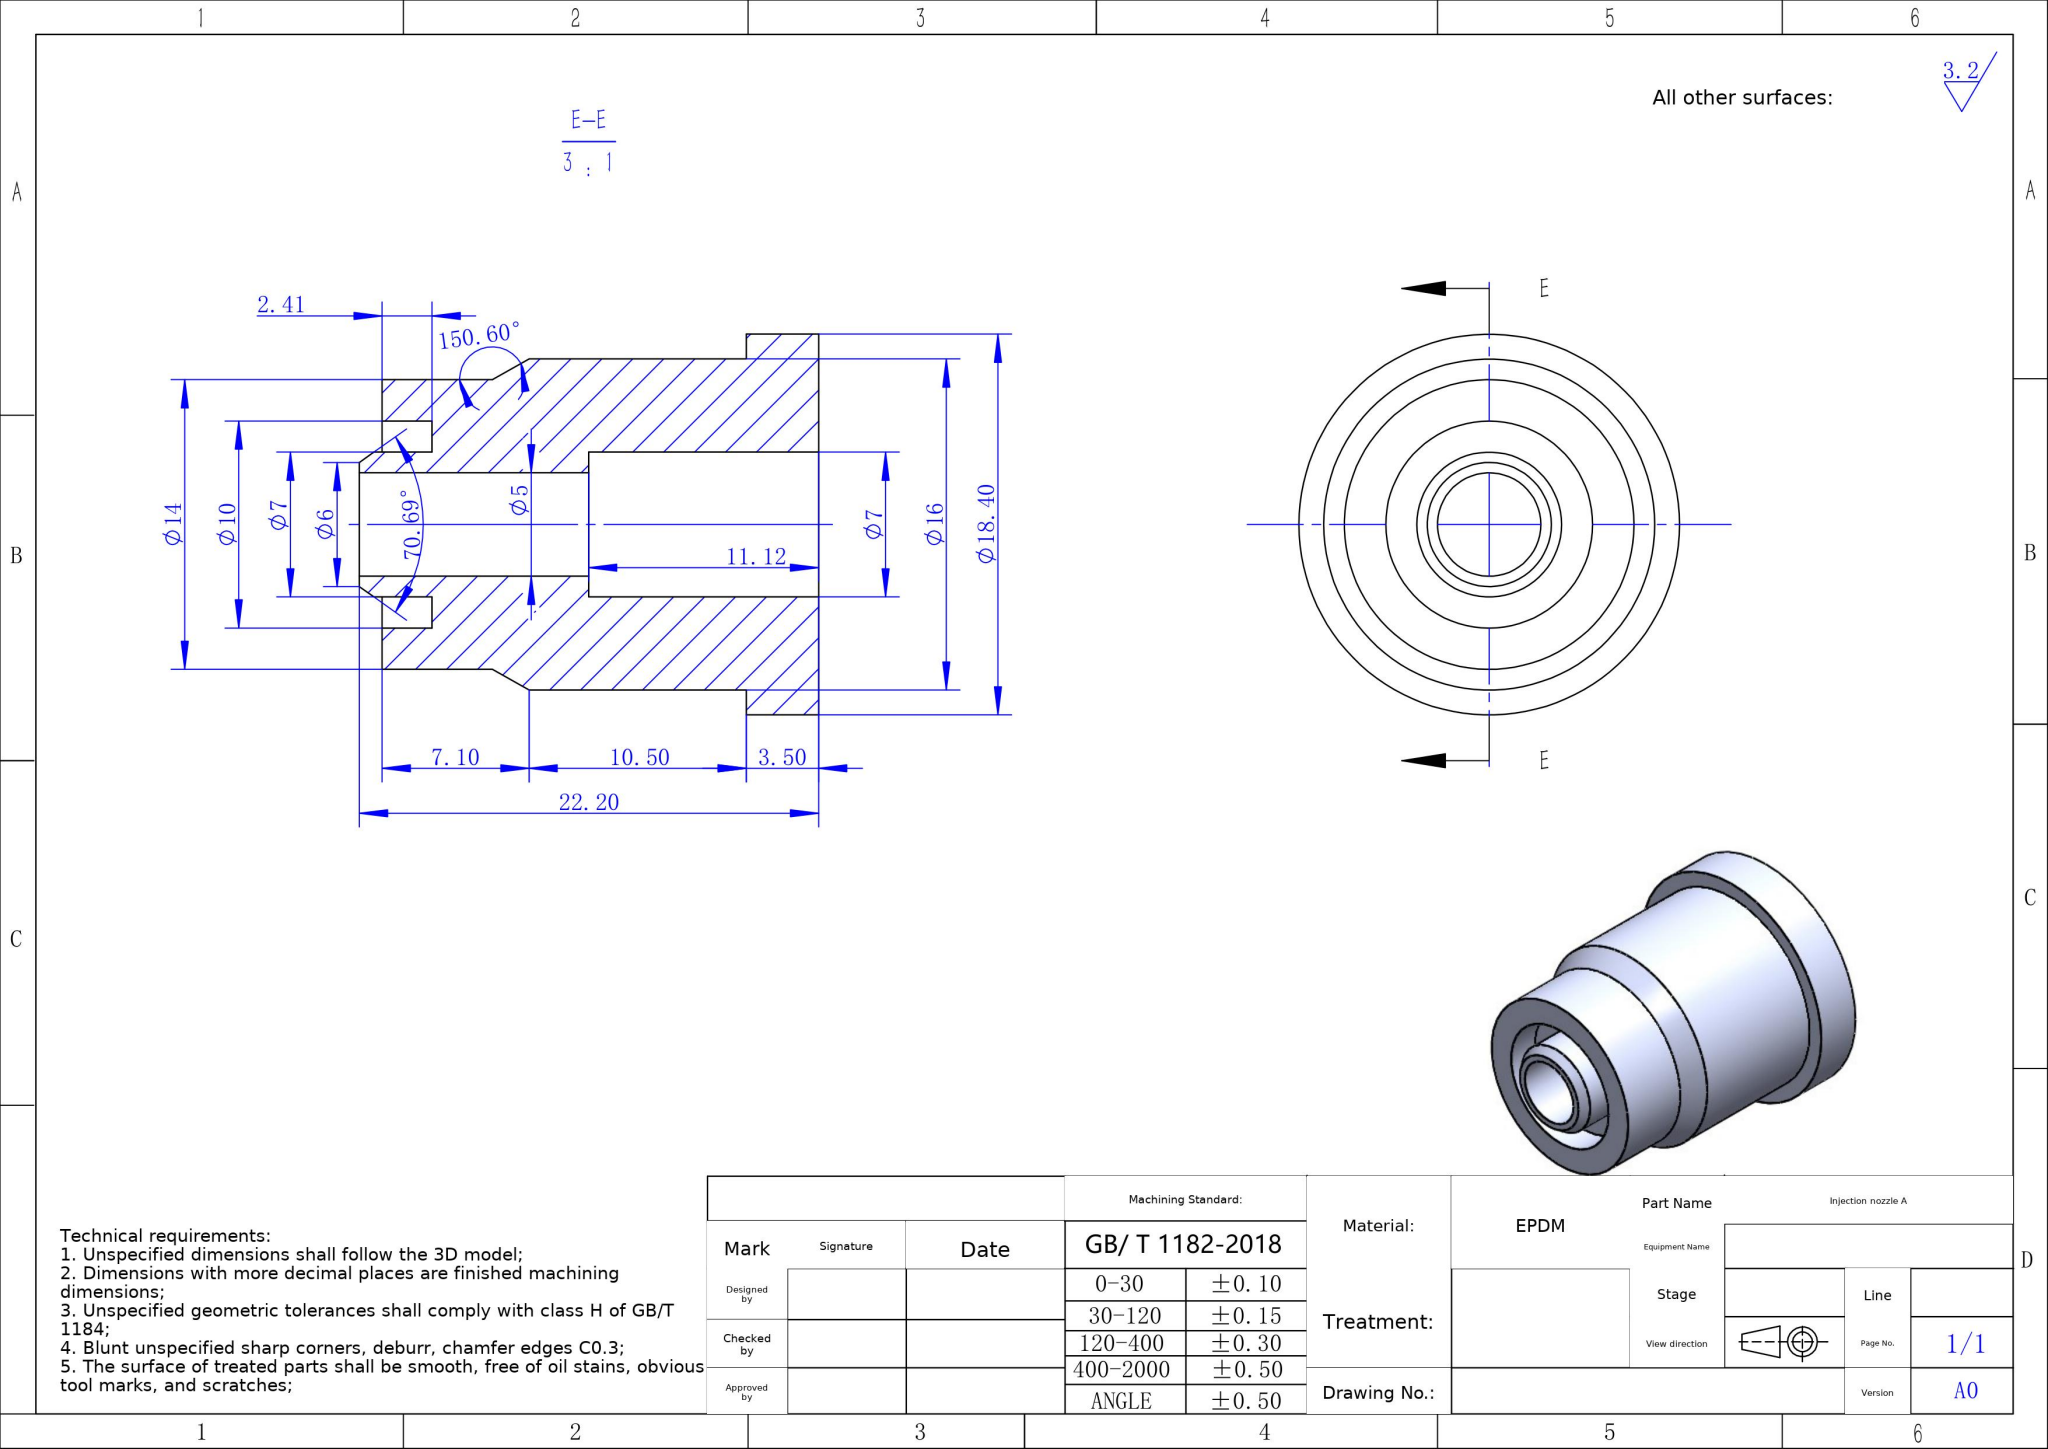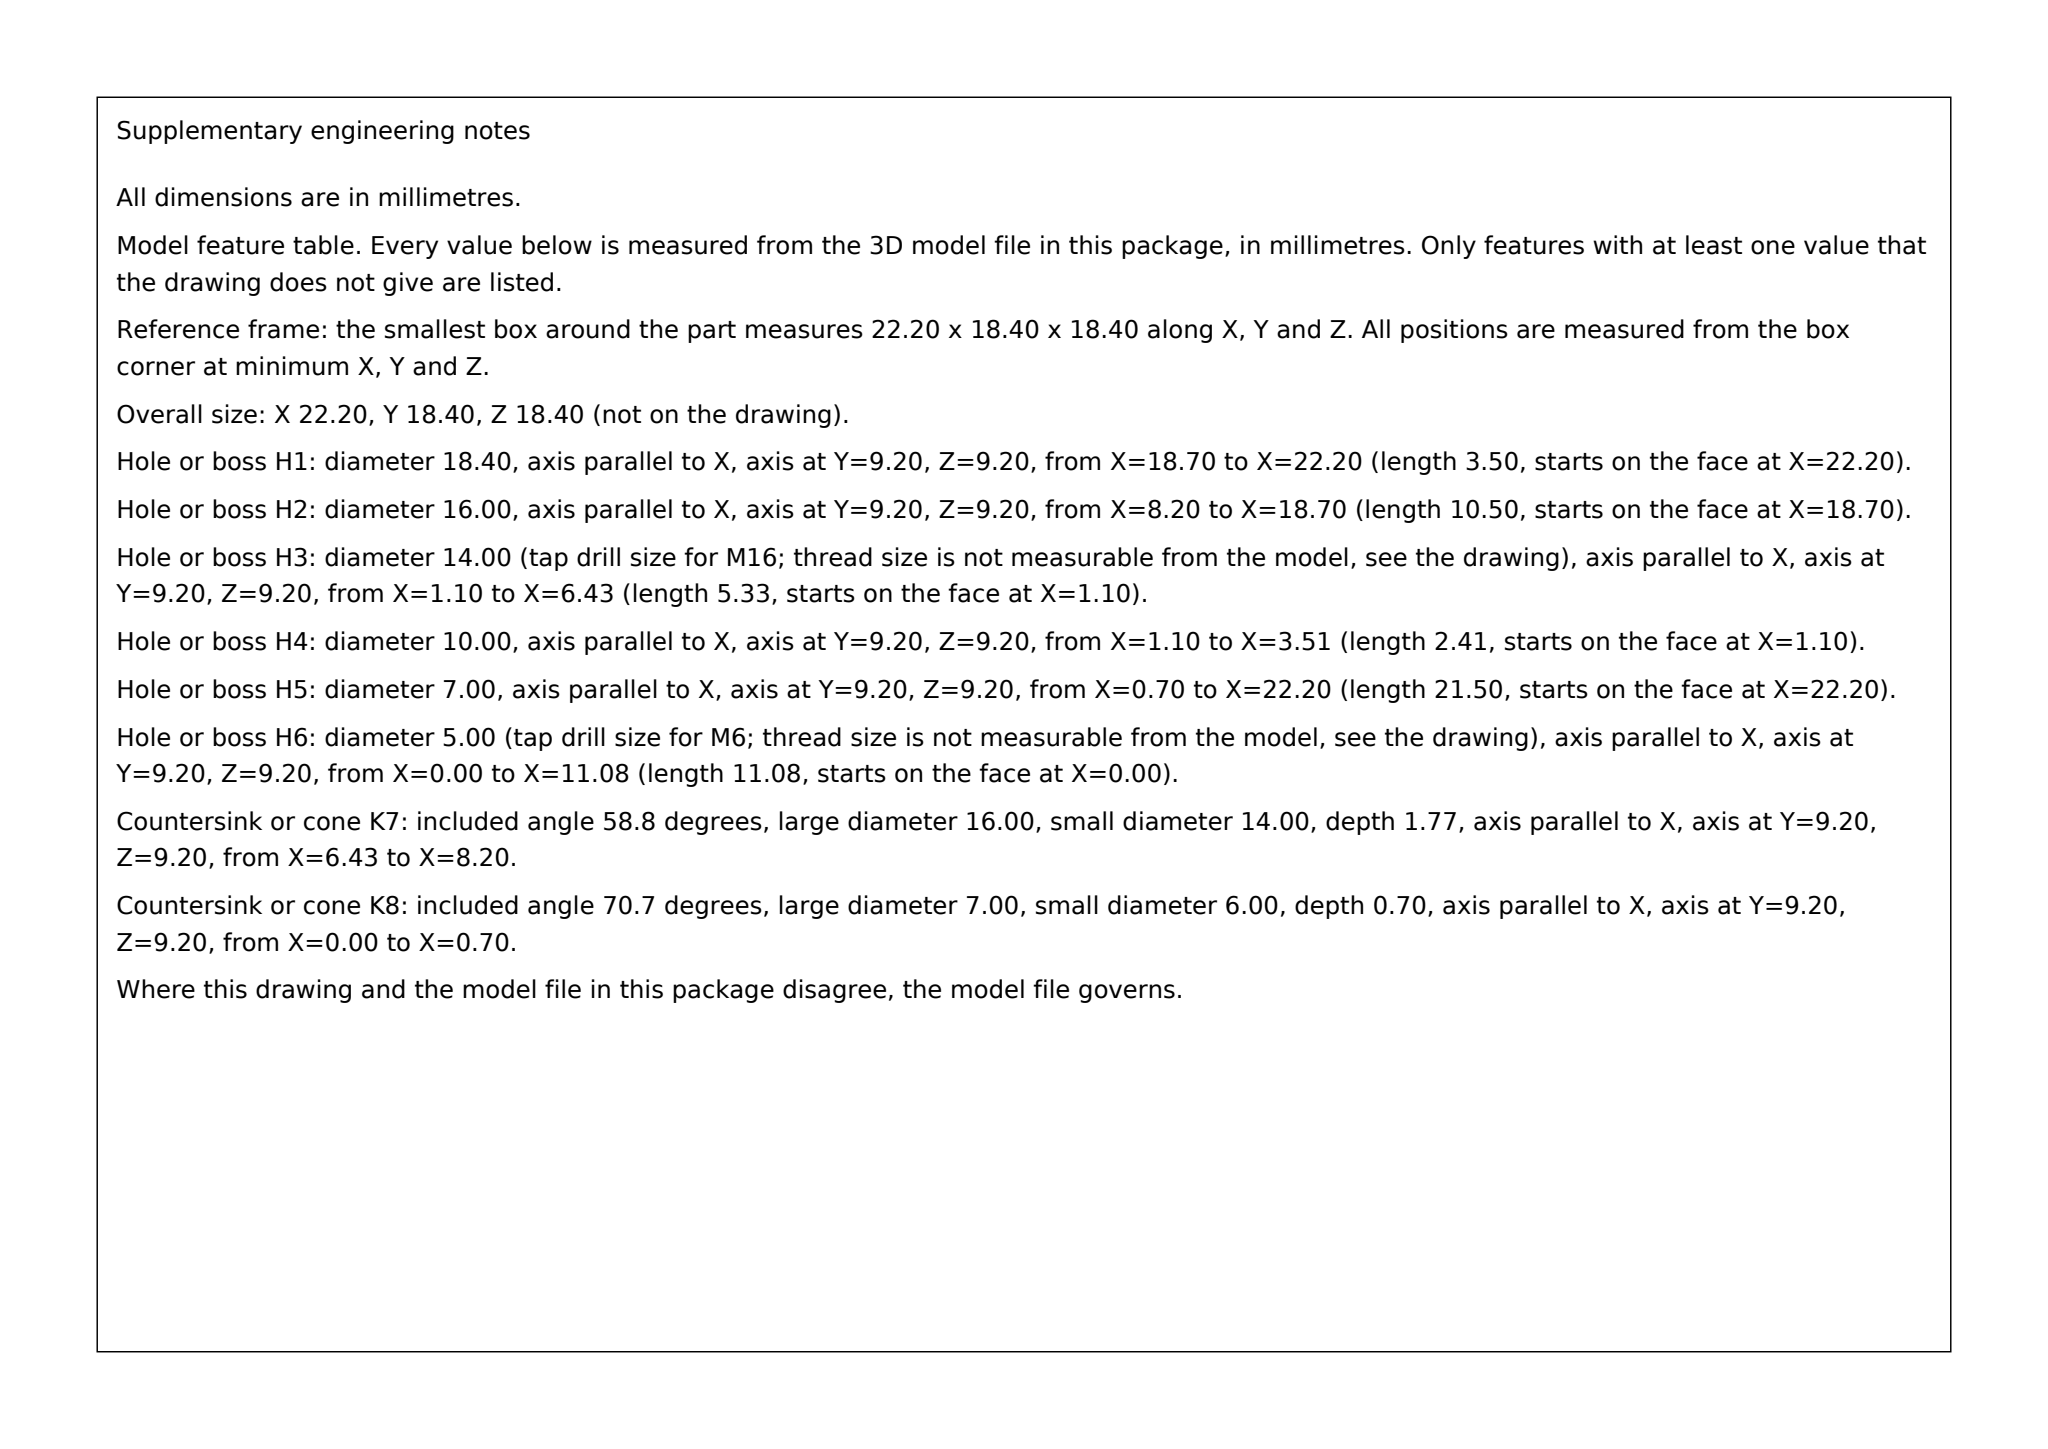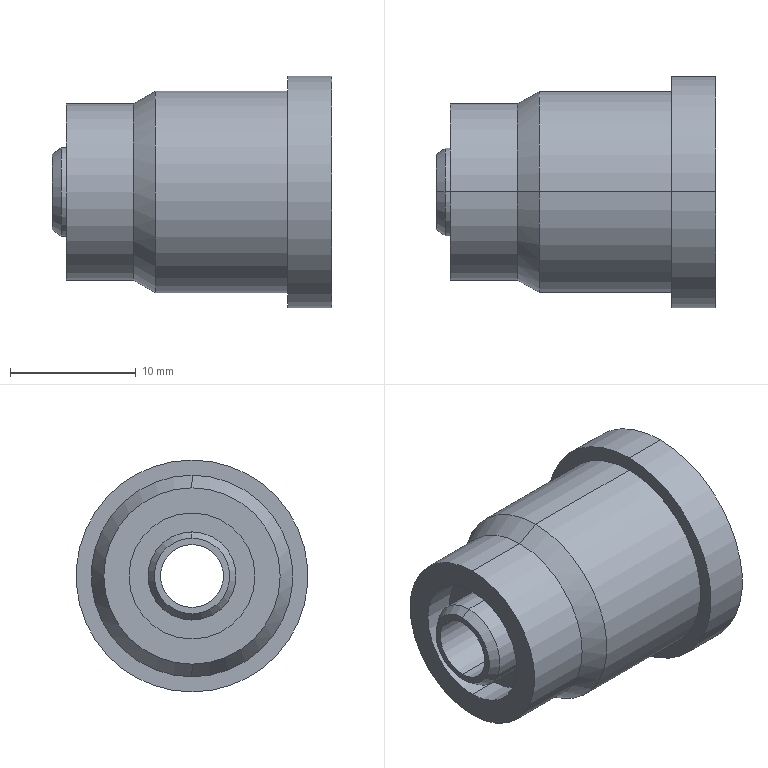Part | SolidWorks | mm | material EPDM | 1 solid | 24 faces | box 22.2 x 18.4 x 18.4 mm | volume 3472 mm3 | cylinder 14 | plane 6 | cone 4 | commonest cylinder face diameters 7 x4 5 x2 10 x2 14 x2 16 x2 18.4 x2
STEP:
#1=CARTESIAN_POINT('',(-32.162,0.,3.));
#2=VERTEX_POINT('',#1);
#3=CARTESIAN_POINT('',(-32.162,0.,-3.));
#4=VERTEX_POINT('',#3);
#5=CARTESIAN_POINT('',(-32.162,0.,0.));
#6=DIRECTION('',(-1.,0.,0.));
#7=DIRECTION('',(0.,0.,1.));
#8=AXIS2_PLACEMENT_3D('',#5,#6,#7);
#9=CIRCLE('',#8,3.);
#10=EDGE_CURVE('',#2,#4,#9,.T.);
#11=ORIENTED_EDGE('',*,*,#10,.F.);
#12=CARTESIAN_POINT('',(-31.457,0.,3.5));
#13=VERTEX_POINT('',#12);
#14=CARTESIAN_POINT('',(-32.162,0.,3.));
#15=DIRECTION('',(0.8157,0.,0.5785));
#16=VECTOR('',#15,1000.);
#17=LINE('',#14,#16);
#18=EDGE_CURVE('',#2,#13,#17,.T.);
#19=ORIENTED_EDGE('',*,*,#18,.T.);
#20=CARTESIAN_POINT('',(-31.457,0.,-3.5));
#21=VERTEX_POINT('',#20);
#22=CARTESIAN_POINT('',(-31.457,0.,0.));
#23=DIRECTION('',(-1.,0.,0.));
#24=DIRECTION('',(0.,0.,-1.));
#25=AXIS2_PLACEMENT_3D('',#22,#23,#24);
#26=CIRCLE('',#25,3.5);
#27=EDGE_CURVE('',#13,#21,#26,.T.);
#28=ORIENTED_EDGE('',*,*,#27,.T.);
#29=CARTESIAN_POINT('',(-32.162,0.,-3.));
#30=DIRECTION('',(0.8157,0.,-0.5785));
#31=VECTOR('',#30,1000.);
#32=LINE('',#29,#31);
#33=EDGE_CURVE('',#4,#21,#32,.T.);
#34=ORIENTED_EDGE('',*,*,#33,.F.);
#35=EDGE_LOOP('',(#11,#19,#28,#34));
#36=FACE_OUTER_BOUND('',#35,.T.);
#37=CARTESIAN_POINT('',(-32.162,0.,0.));
#38=DIRECTION('',(1.,0.,0.));
#39=DIRECTION('',(0.,0.,-1.));
#40=AXIS2_PLACEMENT_3D('',#37,#38,#39);
#41=CONICAL_SURFACE('',#40,3.,0.6169);
#42=ADVANCED_FACE('',(#36),#41,.T.);
#43=CARTESIAN_POINT('',(-9.962,0.,-3.5));
#44=VERTEX_POINT('',#43);
#45=CARTESIAN_POINT('',(-9.962,0.,3.5));
#46=VERTEX_POINT('',#45);
#47=CARTESIAN_POINT('',(-9.962,0.,0.));
#48=DIRECTION('',(-1.,0.,0.));
#49=DIRECTION('',(0.,0.,1.));
#50=AXIS2_PLACEMENT_3D('',#47,#48,#49);
#51=CIRCLE('',#50,3.5);
#52=EDGE_CURVE('',#44,#46,#51,.T.);
#53=ORIENTED_EDGE('',*,*,#52,.F.);
#54=CARTESIAN_POINT('',(-21.082,0.,-3.5));
#55=VERTEX_POINT('',#54);
#56=CARTESIAN_POINT('',(-9.9,0.,-3.5));
#57=DIRECTION('',(-1.,0.,0.));
#58=VECTOR('',#57,1000.);
#59=LINE('',#56,#58);
#60=EDGE_CURVE('',#44,#55,#59,.T.);
#61=ORIENTED_EDGE('',*,*,#60,.T.);
#62=CARTESIAN_POINT('',(-21.082,0.,3.5));
#63=VERTEX_POINT('',#62);
#64=CARTESIAN_POINT('',(-21.082,0.,0.));
#65=DIRECTION('',(-1.,0.,0.));
#66=DIRECTION('',(0.,0.,1.));
#67=AXIS2_PLACEMENT_3D('',#64,#65,#66);
#68=CIRCLE('',#67,3.5);
#69=EDGE_CURVE('',#55,#63,#68,.T.);
#70=ORIENTED_EDGE('',*,*,#69,.T.);
#71=CARTESIAN_POINT('',(-9.9,0.,3.5));
#72=DIRECTION('',(-1.,0.,0.));
#73=VECTOR('',#72,1000.);
#74=LINE('',#71,#73);
#75=EDGE_CURVE('',#46,#63,#74,.T.);
#76=ORIENTED_EDGE('',*,*,#75,.F.);
#77=EDGE_LOOP('',(#53,#61,#70,#76));
#78=FACE_OUTER_BOUND('',#77,.T.);
#79=CARTESIAN_POINT('',(-9.9,0.,0.));
#80=DIRECTION('',(-1.,0.,0.));
#81=DIRECTION('',(0.,0.,1.));
#82=AXIS2_PLACEMENT_3D('',#79,#80,#81);
#83=CYLINDRICAL_SURFACE('',#82,3.5);
#84=ADVANCED_FACE('',(#78),#83,.F.);
#85=CARTESIAN_POINT('',(-21.082,0.,-2.5));
#86=VERTEX_POINT('',#85);
#87=CARTESIAN_POINT('',(-21.082,0.,2.5));
#88=VERTEX_POINT('',#87);
#89=CARTESIAN_POINT('',(-21.082,0.,0.));
#90=DIRECTION('',(-1.,0.,0.));
#91=DIRECTION('',(0.,0.,1.));
#92=AXIS2_PLACEMENT_3D('',#89,#90,#91);
#93=CIRCLE('',#92,2.5);
#94=EDGE_CURVE('',#86,#88,#93,.T.);
#95=ORIENTED_EDGE('',*,*,#94,.F.);
#96=CARTESIAN_POINT('',(-32.162,0.,-2.5));
#97=VERTEX_POINT('',#96);
#98=CARTESIAN_POINT('',(-9.9,0.,-2.5));
#99=DIRECTION('',(-1.,0.,0.));
#100=VECTOR('',#99,1000.);
#101=LINE('',#98,#100);
#102=EDGE_CURVE('',#86,#97,#101,.T.);
#103=ORIENTED_EDGE('',*,*,#102,.T.);
#104=CARTESIAN_POINT('',(-32.162,0.,2.5));
#105=VERTEX_POINT('',#104);
#106=CARTESIAN_POINT('',(-32.162,0.,0.));
#107=DIRECTION('',(-1.,0.,0.));
#108=DIRECTION('',(0.,0.,1.));
#109=AXIS2_PLACEMENT_3D('',#106,#107,#108);
#110=CIRCLE('',#109,2.5);
#111=EDGE_CURVE('',#97,#105,#110,.T.);
#112=ORIENTED_EDGE('',*,*,#111,.T.);
#113=CARTESIAN_POINT('',(-9.9,0.,2.5));
#114=DIRECTION('',(-1.,0.,0.));
#115=VECTOR('',#114,1000.);
#116=LINE('',#113,#115);
#117=EDGE_CURVE('',#88,#105,#116,.T.);
#118=ORIENTED_EDGE('',*,*,#117,.F.);
#119=EDGE_LOOP('',(#95,#103,#112,#118));
#120=FACE_OUTER_BOUND('',#119,.T.);
#121=CARTESIAN_POINT('',(-9.9,0.,0.));
#122=DIRECTION('',(-1.,0.,0.));
#123=DIRECTION('',(0.,0.,1.));
#124=AXIS2_PLACEMENT_3D('',#121,#122,#123);
#125=CYLINDRICAL_SURFACE('',#124,2.5);
#126=ADVANCED_FACE('',(#120),#125,.F.);
#127=CARTESIAN_POINT('',(-28.652,0.,-5.));
#128=VERTEX_POINT('',#127);
#129=CARTESIAN_POINT('',(-28.652,0.,5.));
#130=VERTEX_POINT('',#129);
#131=CARTESIAN_POINT('',(-28.652,0.,0.));
#132=DIRECTION('',(-1.,0.,0.));
#133=DIRECTION('',(0.,0.,1.));
#134=AXIS2_PLACEMENT_3D('',#131,#132,#133);
#135=CIRCLE('',#134,5.);
#136=EDGE_CURVE('',#128,#130,#135,.T.);
#137=ORIENTED_EDGE('',*,*,#136,.F.);
#138=CARTESIAN_POINT('',(-31.062,0.,-5.));
#139=VERTEX_POINT('',#138);
#140=CARTESIAN_POINT('',(-9.9,0.,-5.));
#141=DIRECTION('',(-1.,0.,0.));
#142=VECTOR('',#141,1000.);
#143=LINE('',#140,#142);
#144=EDGE_CURVE('',#128,#139,#143,.T.);
#145=ORIENTED_EDGE('',*,*,#144,.T.);
#146=CARTESIAN_POINT('',(-31.062,0.,5.));
#147=VERTEX_POINT('',#146);
#148=CARTESIAN_POINT('',(-31.062,0.,0.));
#149=DIRECTION('',(-1.,0.,0.));
#150=DIRECTION('',(0.,0.,1.));
#151=AXIS2_PLACEMENT_3D('',#148,#149,#150);
#152=CIRCLE('',#151,5.);
#153=EDGE_CURVE('',#139,#147,#152,.T.);
#154=ORIENTED_EDGE('',*,*,#153,.T.);
#155=CARTESIAN_POINT('',(-9.9,0.,5.));
#156=DIRECTION('',(-1.,0.,0.));
#157=VECTOR('',#156,1000.);
#158=LINE('',#155,#157);
#159=EDGE_CURVE('',#130,#147,#158,.T.);
#160=ORIENTED_EDGE('',*,*,#159,.F.);
#161=EDGE_LOOP('',(#137,#145,#154,#160));
#162=FACE_OUTER_BOUND('',#161,.T.);
#163=CARTESIAN_POINT('',(-9.9,0.,0.));
#164=DIRECTION('',(-1.,0.,0.));
#165=DIRECTION('',(0.,0.,1.));
#166=AXIS2_PLACEMENT_3D('',#163,#164,#165);
#167=CYLINDRICAL_SURFACE('',#166,5.);
#168=ADVANCED_FACE('',(#162),#167,.F.);
#169=CARTESIAN_POINT('',(-25.737,0.,7.));
#170=VERTEX_POINT('',#169);
#171=CARTESIAN_POINT('',(-25.737,0.,-7.));
#172=VERTEX_POINT('',#171);
#173=CARTESIAN_POINT('',(-25.737,0.,0.));
#174=DIRECTION('',(-1.,0.,0.));
#175=DIRECTION('',(0.,0.,1.));
#176=AXIS2_PLACEMENT_3D('',#173,#174,#175);
#177=CIRCLE('',#176,7.);
#178=EDGE_CURVE('',#170,#172,#177,.T.);
#179=ORIENTED_EDGE('',*,*,#178,.T.);
#180=CARTESIAN_POINT('',(-31.062,0.,-7.));
#181=VERTEX_POINT('',#180);
#182=CARTESIAN_POINT('',(-9.9,0.,-7.));
#183=DIRECTION('',(-1.,0.,0.));
#184=VECTOR('',#183,1000.);
#185=LINE('',#182,#184);
#186=EDGE_CURVE('',#172,#181,#185,.T.);
#187=ORIENTED_EDGE('',*,*,#186,.T.);
#188=CARTESIAN_POINT('',(-31.062,0.,7.));
#189=VERTEX_POINT('',#188);
#190=CARTESIAN_POINT('',(-31.062,0.,0.));
#191=DIRECTION('',(-1.,0.,0.));
#192=DIRECTION('',(0.,0.,1.));
#193=AXIS2_PLACEMENT_3D('',#190,#191,#192);
#194=CIRCLE('',#193,7.);
#195=EDGE_CURVE('',#189,#181,#194,.T.);
#196=ORIENTED_EDGE('',*,*,#195,.F.);
#197=CARTESIAN_POINT('',(-9.9,0.,7.));
#198=DIRECTION('',(-1.,0.,0.));
#199=VECTOR('',#198,1000.);
#200=LINE('',#197,#199);
#201=EDGE_CURVE('',#170,#189,#200,.T.);
#202=ORIENTED_EDGE('',*,*,#201,.F.);
#203=EDGE_LOOP('',(#179,#187,#196,#202));
#204=FACE_OUTER_BOUND('',#203,.T.);
#205=CARTESIAN_POINT('',(-9.9,0.,0.));
#206=DIRECTION('',(-1.,0.,0.));
#207=DIRECTION('',(0.,0.,1.));
#208=AXIS2_PLACEMENT_3D('',#205,#206,#207);
#209=CYLINDRICAL_SURFACE('',#208,7.);
#210=ADVANCED_FACE('',(#204),#209,.T.);
#211=ORIENTED_EDGE('',*,*,#178,.F.);
#212=CARTESIAN_POINT('',(-23.962,0.,8.));
#213=VERTEX_POINT('',#212);
#214=CARTESIAN_POINT('',(-23.962,0.,8.));
#215=DIRECTION('',(0.8712,0.,0.4909));
#216=VECTOR('',#215,1000.);
#217=LINE('',#214,#216);
#218=EDGE_CURVE('',#170,#213,#217,.T.);
#219=ORIENTED_EDGE('',*,*,#218,.T.);
#220=CARTESIAN_POINT('',(-23.962,0.,-8.));
#221=VERTEX_POINT('',#220);
#222=CARTESIAN_POINT('',(-23.962,0.,0.));
#223=DIRECTION('',(-1.,0.,0.));
#224=DIRECTION('',(0.,0.,1.));
#225=AXIS2_PLACEMENT_3D('',#222,#223,#224);
#226=CIRCLE('',#225,8.);
#227=EDGE_CURVE('',#213,#221,#226,.T.);
#228=ORIENTED_EDGE('',*,*,#227,.T.);
#229=CARTESIAN_POINT('',(-23.962,0.,-8.));
#230=DIRECTION('',(0.8712,0.,-0.4909));
#231=VECTOR('',#230,1000.);
#232=LINE('',#229,#231);
#233=EDGE_CURVE('',#172,#221,#232,.T.);
#234=ORIENTED_EDGE('',*,*,#233,.F.);
#235=EDGE_LOOP('',(#211,#219,#228,#234));
#236=FACE_OUTER_BOUND('',#235,.T.);
#237=CARTESIAN_POINT('',(-23.962,0.,0.));
#238=DIRECTION('',(1.,0.,0.));
#239=DIRECTION('',(0.,0.,-1.));
#240=AXIS2_PLACEMENT_3D('',#237,#238,#239);
#241=CONICAL_SURFACE('',#240,8.,0.5131);
#242=ADVANCED_FACE('',(#236),#241,.T.);
#243=CARTESIAN_POINT('',(-13.462,0.,8.));
#244=VERTEX_POINT('',#243);
#245=CARTESIAN_POINT('',(-13.462,0.,-8.));
#246=VERTEX_POINT('',#245);
#247=CARTESIAN_POINT('',(-13.462,0.,0.));
#248=DIRECTION('',(-1.,0.,0.));
#249=DIRECTION('',(0.,0.,1.));
#250=AXIS2_PLACEMENT_3D('',#247,#248,#249);
#251=CIRCLE('',#250,8.);
#252=EDGE_CURVE('',#244,#246,#251,.T.);
#253=ORIENTED_EDGE('',*,*,#252,.T.);
#254=CARTESIAN_POINT('',(-9.9,0.,-8.));
#255=DIRECTION('',(-1.,0.,0.));
#256=VECTOR('',#255,1000.);
#257=LINE('',#254,#256);
#258=EDGE_CURVE('',#246,#221,#257,.T.);
#259=ORIENTED_EDGE('',*,*,#258,.T.);
#260=ORIENTED_EDGE('',*,*,#227,.F.);
#261=CARTESIAN_POINT('',(-9.9,0.,8.));
#262=DIRECTION('',(-1.,0.,0.));
#263=VECTOR('',#262,1000.);
#264=LINE('',#261,#263);
#265=EDGE_CURVE('',#244,#213,#264,.T.);
#266=ORIENTED_EDGE('',*,*,#265,.F.);
#267=EDGE_LOOP('',(#253,#259,#260,#266));
#268=FACE_OUTER_BOUND('',#267,.T.);
#269=CARTESIAN_POINT('',(-9.9,0.,0.));
#270=DIRECTION('',(-1.,0.,0.));
#271=DIRECTION('',(0.,0.,1.));
#272=AXIS2_PLACEMENT_3D('',#269,#270,#271);
#273=CYLINDRICAL_SURFACE('',#272,8.);
#274=ADVANCED_FACE('',(#268),#273,.T.);
#275=CARTESIAN_POINT('',(-9.962,0.,9.2));
#276=VERTEX_POINT('',#275);
#277=CARTESIAN_POINT('',(-9.962,0.,-9.2));
#278=VERTEX_POINT('',#277);
#279=CARTESIAN_POINT('',(-9.962,0.,0.));
#280=DIRECTION('',(-1.,0.,0.));
#281=DIRECTION('',(0.,0.,1.));
#282=AXIS2_PLACEMENT_3D('',#279,#280,#281);
#283=CIRCLE('',#282,9.2);
#284=EDGE_CURVE('',#276,#278,#283,.T.);
#285=ORIENTED_EDGE('',*,*,#284,.T.);
#286=CARTESIAN_POINT('',(-13.462,0.,-9.2));
#287=VERTEX_POINT('',#286);
#288=CARTESIAN_POINT('',(-9.9,0.,-9.2));
#289=DIRECTION('',(-1.,0.,0.));
#290=VECTOR('',#289,1000.);
#291=LINE('',#288,#290);
#292=EDGE_CURVE('',#278,#287,#291,.T.);
#293=ORIENTED_EDGE('',*,*,#292,.T.);
#294=CARTESIAN_POINT('',(-13.462,0.,9.2));
#295=VERTEX_POINT('',#294);
#296=CARTESIAN_POINT('',(-13.462,0.,0.));
#297=DIRECTION('',(-1.,0.,0.));
#298=DIRECTION('',(0.,0.,1.));
#299=AXIS2_PLACEMENT_3D('',#296,#297,#298);
#300=CIRCLE('',#299,9.2);
#301=EDGE_CURVE('',#295,#287,#300,.T.);
#302=ORIENTED_EDGE('',*,*,#301,.F.);
#303=CARTESIAN_POINT('',(-9.9,0.,9.2));
#304=DIRECTION('',(-1.,0.,0.));
#305=VECTOR('',#304,1000.);
#306=LINE('',#303,#305);
#307=EDGE_CURVE('',#276,#295,#306,.T.);
#308=ORIENTED_EDGE('',*,*,#307,.F.);
#309=EDGE_LOOP('',(#285,#293,#302,#308));
#310=FACE_OUTER_BOUND('',#309,.T.);
#311=CARTESIAN_POINT('',(-9.9,0.,0.));
#312=DIRECTION('',(-1.,0.,0.));
#313=DIRECTION('',(0.,0.,1.));
#314=AXIS2_PLACEMENT_3D('',#311,#312,#313);
#315=CYLINDRICAL_SURFACE('',#314,9.2);
#316=ADVANCED_FACE('',(#310),#315,.T.);
#317=CARTESIAN_POINT('',(-28.652,0.,3.5));
#318=VERTEX_POINT('',#317);
#319=CARTESIAN_POINT('',(-28.652,0.,-3.5));
#320=VERTEX_POINT('',#319);
#321=CARTESIAN_POINT('',(-28.652,0.,0.));
#322=DIRECTION('',(-1.,0.,0.));
#323=DIRECTION('',(0.,0.,1.));
#324=AXIS2_PLACEMENT_3D('',#321,#322,#323);
#325=CIRCLE('',#324,3.5);
#326=EDGE_CURVE('',#318,#320,#325,.T.);
#327=ORIENTED_EDGE('',*,*,#326,.T.);
#328=CARTESIAN_POINT('',(-9.9,0.,-3.5));
#329=DIRECTION('',(-1.,0.,0.));
#330=VECTOR('',#329,1000.);
#331=LINE('',#328,#330);
#332=EDGE_CURVE('',#320,#21,#331,.T.);
#333=ORIENTED_EDGE('',*,*,#332,.T.);
#334=ORIENTED_EDGE('',*,*,#27,.F.);
#335=CARTESIAN_POINT('',(-9.9,0.,3.5));
#336=DIRECTION('',(-1.,0.,0.));
#337=VECTOR('',#336,1000.);
#338=LINE('',#335,#337);
#339=EDGE_CURVE('',#318,#13,#338,.T.);
#340=ORIENTED_EDGE('',*,*,#339,.F.);
#341=EDGE_LOOP('',(#327,#333,#334,#340));
#342=FACE_OUTER_BOUND('',#341,.T.);
#343=CARTESIAN_POINT('',(-9.9,0.,0.));
#344=DIRECTION('',(-1.,0.,0.));
#345=DIRECTION('',(0.,0.,1.));
#346=AXIS2_PLACEMENT_3D('',#343,#344,#345);
#347=CYLINDRICAL_SURFACE('',#346,3.5);
#348=ADVANCED_FACE('',(#342),#347,.T.);
#349=ORIENTED_EDGE('',*,*,#332,.F.);
#350=CARTESIAN_POINT('',(-28.652,0.,0.));
#351=DIRECTION('',(-1.,0.,0.));
#352=DIRECTION('',(0.,0.,1.));
#353=AXIS2_PLACEMENT_3D('',#350,#351,#352);
#354=CIRCLE('',#353,3.5);
#355=EDGE_CURVE('',#320,#318,#354,.T.);
#356=ORIENTED_EDGE('',*,*,#355,.T.);
#357=ORIENTED_EDGE('',*,*,#339,.T.);
#358=CARTESIAN_POINT('',(-31.457,0.,0.));
#359=DIRECTION('',(-1.,0.,0.));
#360=DIRECTION('',(0.,0.,-1.));
#361=AXIS2_PLACEMENT_3D('',#358,#359,#360);
#362=CIRCLE('',#361,3.5);
#363=EDGE_CURVE('',#21,#13,#362,.T.);
#364=ORIENTED_EDGE('',*,*,#363,.F.);
#365=EDGE_LOOP('',(#349,#356,#357,#364));
#366=FACE_OUTER_BOUND('',#365,.T.);
#367=CARTESIAN_POINT('',(-9.9,0.,0.));
#368=DIRECTION('',(-1.,0.,0.));
#369=DIRECTION('',(0.,0.,1.));
#370=AXIS2_PLACEMENT_3D('',#367,#368,#369);
#371=CYLINDRICAL_SURFACE('',#370,3.5);
#372=ADVANCED_FACE('',(#366),#371,.T.);
#373=CARTESIAN_POINT('',(-32.162,0.,0.));
#374=DIRECTION('',(-1.,0.,0.));
#375=DIRECTION('',(0.,0.,1.));
#376=AXIS2_PLACEMENT_3D('',#373,#374,#375);
#377=CIRCLE('',#376,2.5);
#378=EDGE_CURVE('',#105,#97,#377,.T.);
#379=ORIENTED_EDGE('',*,*,#378,.F.);
#380=ORIENTED_EDGE('',*,*,#111,.F.);
#381=EDGE_LOOP('',(#379,#380));
#382=FACE_BOUND('',#381,.T.);
#383=CARTESIAN_POINT('',(-32.162,0.,0.));
#384=DIRECTION('',(-1.,0.,0.));
#385=DIRECTION('',(0.,0.,1.));
#386=AXIS2_PLACEMENT_3D('',#383,#384,#385);
#387=CIRCLE('',#386,3.);
#388=EDGE_CURVE('',#4,#2,#387,.T.);
#389=ORIENTED_EDGE('',*,*,#388,.T.);
#390=ORIENTED_EDGE('',*,*,#10,.T.);
#391=EDGE_LOOP('',(#389,#390));
#392=FACE_OUTER_BOUND('',#391,.T.);
#393=CARTESIAN_POINT('',(-32.162,3.5,0.));
#394=DIRECTION('',(1.,0.,0.));
#395=DIRECTION('',(0.,0.,-1.));
#396=AXIS2_PLACEMENT_3D('',#393,#394,#395);
#397=PLANE('',#396);
#398=ADVANCED_FACE('',(#382,#392),#397,.F.);
#399=ORIENTED_EDGE('',*,*,#292,.F.);
#400=CARTESIAN_POINT('',(-9.962,0.,0.));
#401=DIRECTION('',(-1.,0.,0.));
#402=DIRECTION('',(0.,0.,1.));
#403=AXIS2_PLACEMENT_3D('',#400,#401,#402);
#404=CIRCLE('',#403,9.2);
#405=EDGE_CURVE('',#278,#276,#404,.T.);
#406=ORIENTED_EDGE('',*,*,#405,.T.);
#407=ORIENTED_EDGE('',*,*,#307,.T.);
#408=CARTESIAN_POINT('',(-13.462,0.,0.));
#409=DIRECTION('',(-1.,0.,0.));
#410=DIRECTION('',(0.,0.,1.));
#411=AXIS2_PLACEMENT_3D('',#408,#409,#410);
#412=CIRCLE('',#411,9.2);
#413=EDGE_CURVE('',#287,#295,#412,.T.);
#414=ORIENTED_EDGE('',*,*,#413,.F.);
#415=EDGE_LOOP('',(#399,#406,#407,#414));
#416=FACE_OUTER_BOUND('',#415,.T.);
#417=CARTESIAN_POINT('',(-9.9,0.,0.));
#418=DIRECTION('',(-1.,0.,0.));
#419=DIRECTION('',(0.,0.,1.));
#420=AXIS2_PLACEMENT_3D('',#417,#418,#419);
#421=CYLINDRICAL_SURFACE('',#420,9.2);
#422=ADVANCED_FACE('',(#416),#421,.T.);
#423=ORIENTED_EDGE('',*,*,#252,.F.);
#424=CARTESIAN_POINT('',(-13.462,0.,0.));
#425=DIRECTION('',(-1.,0.,0.));
#426=DIRECTION('',(0.,0.,1.));
#427=AXIS2_PLACEMENT_3D('',#424,#425,#426);
#428=CIRCLE('',#427,8.);
#429=EDGE_CURVE('',#246,#244,#428,.T.);
#430=ORIENTED_EDGE('',*,*,#429,.F.);
#431=EDGE_LOOP('',(#423,#430));
#432=FACE_BOUND('',#431,.T.);
#433=ORIENTED_EDGE('',*,*,#301,.T.);
#434=ORIENTED_EDGE('',*,*,#413,.T.);
#435=EDGE_LOOP('',(#433,#434));
#436=FACE_OUTER_BOUND('',#435,.T.);
#437=CARTESIAN_POINT('',(-13.462,9.2,0.));
#438=DIRECTION('',(1.,0.,0.));
#439=DIRECTION('',(0.,0.,-1.));
#440=AXIS2_PLACEMENT_3D('',#437,#438,#439);
#441=PLANE('',#440);
#442=ADVANCED_FACE('',(#432,#436),#441,.F.);
#443=ORIENTED_EDGE('',*,*,#258,.F.);
#444=ORIENTED_EDGE('',*,*,#429,.T.);
#445=ORIENTED_EDGE('',*,*,#265,.T.);
#446=CARTESIAN_POINT('',(-23.962,0.,0.));
#447=DIRECTION('',(-1.,0.,0.));
#448=DIRECTION('',(0.,0.,1.));
#449=AXIS2_PLACEMENT_3D('',#446,#447,#448);
#450=CIRCLE('',#449,8.);
#451=EDGE_CURVE('',#221,#213,#450,.T.);
#452=ORIENTED_EDGE('',*,*,#451,.F.);
#453=EDGE_LOOP('',(#443,#444,#445,#452));
#454=FACE_OUTER_BOUND('',#453,.T.);
#455=CARTESIAN_POINT('',(-9.9,0.,0.));
#456=DIRECTION('',(-1.,0.,0.));
#457=DIRECTION('',(0.,0.,1.));
#458=AXIS2_PLACEMENT_3D('',#455,#456,#457);
#459=CYLINDRICAL_SURFACE('',#458,8.);
#460=ADVANCED_FACE('',(#454),#459,.T.);
#461=ORIENTED_EDGE('',*,*,#218,.F.);
#462=CARTESIAN_POINT('',(-25.737,0.,0.));
#463=DIRECTION('',(-1.,0.,0.));
#464=DIRECTION('',(0.,0.,1.));
#465=AXIS2_PLACEMENT_3D('',#462,#463,#464);
#466=CIRCLE('',#465,7.);
#467=EDGE_CURVE('',#172,#170,#466,.T.);
#468=ORIENTED_EDGE('',*,*,#467,.F.);
#469=ORIENTED_EDGE('',*,*,#233,.T.);
#470=ORIENTED_EDGE('',*,*,#451,.T.);
#471=EDGE_LOOP('',(#461,#468,#469,#470));
#472=FACE_OUTER_BOUND('',#471,.T.);
#473=CARTESIAN_POINT('',(-23.962,0.,0.));
#474=DIRECTION('',(1.,0.,0.));
#475=DIRECTION('',(0.,0.,-1.));
#476=AXIS2_PLACEMENT_3D('',#473,#474,#475);
#477=CONICAL_SURFACE('',#476,8.,0.5131);
#478=ADVANCED_FACE('',(#472),#477,.T.);
#479=ORIENTED_EDGE('',*,*,#186,.F.);
#480=ORIENTED_EDGE('',*,*,#467,.T.);
#481=ORIENTED_EDGE('',*,*,#201,.T.);
#482=CARTESIAN_POINT('',(-31.062,0.,0.));
#483=DIRECTION('',(-1.,0.,0.));
#484=DIRECTION('',(0.,0.,1.));
#485=AXIS2_PLACEMENT_3D('',#482,#483,#484);
#486=CIRCLE('',#485,7.);
#487=EDGE_CURVE('',#181,#189,#486,.T.);
#488=ORIENTED_EDGE('',*,*,#487,.F.);
#489=EDGE_LOOP('',(#479,#480,#481,#488));
#490=FACE_OUTER_BOUND('',#489,.T.);
#491=CARTESIAN_POINT('',(-9.9,0.,0.));
#492=DIRECTION('',(-1.,0.,0.));
#493=DIRECTION('',(0.,0.,1.));
#494=AXIS2_PLACEMENT_3D('',#491,#492,#493);
#495=CYLINDRICAL_SURFACE('',#494,7.);
#496=ADVANCED_FACE('',(#490),#495,.T.);
#497=CARTESIAN_POINT('',(-31.062,0.,0.));
#498=DIRECTION('',(-1.,0.,0.));
#499=DIRECTION('',(0.,0.,1.));
#500=AXIS2_PLACEMENT_3D('',#497,#498,#499);
#501=CIRCLE('',#500,5.);
#502=EDGE_CURVE('',#147,#139,#501,.T.);
#503=ORIENTED_EDGE('',*,*,#502,.F.);
#504=ORIENTED_EDGE('',*,*,#153,.F.);
#505=EDGE_LOOP('',(#503,#504));
#506=FACE_BOUND('',#505,.T.);
#507=ORIENTED_EDGE('',*,*,#195,.T.);
#508=ORIENTED_EDGE('',*,*,#487,.T.);
#509=EDGE_LOOP('',(#507,#508));
#510=FACE_OUTER_BOUND('',#509,.T.);
#511=CARTESIAN_POINT('',(-31.062,7.,0.));
#512=DIRECTION('',(1.,0.,0.));
#513=DIRECTION('',(0.,0.,-1.));
#514=AXIS2_PLACEMENT_3D('',#511,#512,#513);
#515=PLANE('',#514);
#516=ADVANCED_FACE('',(#506,#510),#515,.F.);
#517=ORIENTED_EDGE('',*,*,#144,.F.);
#518=CARTESIAN_POINT('',(-28.652,0.,0.));
#519=DIRECTION('',(-1.,0.,0.));
#520=DIRECTION('',(0.,0.,1.));
#521=AXIS2_PLACEMENT_3D('',#518,#519,#520);
#522=CIRCLE('',#521,5.);
#523=EDGE_CURVE('',#130,#128,#522,.T.);
#524=ORIENTED_EDGE('',*,*,#523,.F.);
#525=ORIENTED_EDGE('',*,*,#159,.T.);
#526=ORIENTED_EDGE('',*,*,#502,.T.);
#527=EDGE_LOOP('',(#517,#524,#525,#526));
#528=FACE_OUTER_BOUND('',#527,.T.);
#529=CARTESIAN_POINT('',(-9.9,0.,0.));
#530=DIRECTION('',(-1.,0.,0.));
#531=DIRECTION('',(0.,0.,1.));
#532=AXIS2_PLACEMENT_3D('',#529,#530,#531);
#533=CYLINDRICAL_SURFACE('',#532,5.);
#534=ADVANCED_FACE('',(#528),#533,.F.);
#535=ORIENTED_EDGE('',*,*,#326,.F.);
#536=ORIENTED_EDGE('',*,*,#355,.F.);
#537=EDGE_LOOP('',(#535,#536));
#538=FACE_BOUND('',#537,.T.);
#539=ORIENTED_EDGE('',*,*,#523,.T.);
#540=ORIENTED_EDGE('',*,*,#136,.T.);
#541=EDGE_LOOP('',(#539,#540));
#542=FACE_OUTER_BOUND('',#541,.T.);
#543=CARTESIAN_POINT('',(-28.652,5.,0.));
#544=DIRECTION('',(1.,0.,0.));
#545=DIRECTION('',(0.,0.,-1.));
#546=AXIS2_PLACEMENT_3D('',#543,#544,#545);
#547=PLANE('',#546);
#548=ADVANCED_FACE('',(#538,#542),#547,.F.);
#549=ORIENTED_EDGE('',*,*,#102,.F.);
#550=CARTESIAN_POINT('',(-21.082,0.,0.));
#551=DIRECTION('',(-1.,0.,0.));
#552=DIRECTION('',(0.,0.,1.));
#553=AXIS2_PLACEMENT_3D('',#550,#551,#552);
#554=CIRCLE('',#553,2.5);
#555=EDGE_CURVE('',#88,#86,#554,.T.);
#556=ORIENTED_EDGE('',*,*,#555,.F.);
#557=ORIENTED_EDGE('',*,*,#117,.T.);
#558=ORIENTED_EDGE('',*,*,#378,.T.);
#559=EDGE_LOOP('',(#549,#556,#557,#558));
#560=FACE_OUTER_BOUND('',#559,.T.);
#561=CARTESIAN_POINT('',(-9.9,0.,0.));
#562=DIRECTION('',(-1.,0.,0.));
#563=DIRECTION('',(0.,0.,1.));
#564=AXIS2_PLACEMENT_3D('',#561,#562,#563);
#565=CYLINDRICAL_SURFACE('',#564,2.5);
#566=ADVANCED_FACE('',(#560),#565,.F.);
#567=CARTESIAN_POINT('',(-21.082,0.,0.));
#568=DIRECTION('',(-1.,0.,0.));
#569=DIRECTION('',(0.,0.,1.));
#570=AXIS2_PLACEMENT_3D('',#567,#568,#569);
#571=CIRCLE('',#570,3.5);
#572=EDGE_CURVE('',#63,#55,#571,.T.);
#573=ORIENTED_EDGE('',*,*,#572,.F.);
#574=ORIENTED_EDGE('',*,*,#69,.F.);
#575=EDGE_LOOP('',(#573,#574));
#576=FACE_OUTER_BOUND('',#575,.T.);
#577=ORIENTED_EDGE('',*,*,#555,.T.);
#578=ORIENTED_EDGE('',*,*,#94,.T.);
#579=EDGE_LOOP('',(#577,#578));
#580=FACE_BOUND('',#579,.T.);
#581=CARTESIAN_POINT('',(-21.082,2.5,0.));
#582=DIRECTION('',(-1.,0.,0.));
#583=DIRECTION('',(0.,0.,1.));
#584=AXIS2_PLACEMENT_3D('',#581,#582,#583);
#585=PLANE('',#584);
#586=ADVANCED_FACE('',(#576,#580),#585,.F.);
#587=ORIENTED_EDGE('',*,*,#60,.F.);
#588=CARTESIAN_POINT('',(-9.962,0.,0.));
#589=DIRECTION('',(-1.,0.,0.));
#590=DIRECTION('',(0.,0.,1.));
#591=AXIS2_PLACEMENT_3D('',#588,#589,#590);
#592=CIRCLE('',#591,3.5);
#593=EDGE_CURVE('',#46,#44,#592,.T.);
#594=ORIENTED_EDGE('',*,*,#593,.F.);
#595=ORIENTED_EDGE('',*,*,#75,.T.);
#596=ORIENTED_EDGE('',*,*,#572,.T.);
#597=EDGE_LOOP('',(#587,#594,#595,#596));
#598=FACE_OUTER_BOUND('',#597,.T.);
#599=CARTESIAN_POINT('',(-9.9,0.,0.));
#600=DIRECTION('',(-1.,0.,0.));
#601=DIRECTION('',(0.,0.,1.));
#602=AXIS2_PLACEMENT_3D('',#599,#600,#601);
#603=CYLINDRICAL_SURFACE('',#602,3.5);
#604=ADVANCED_FACE('',(#598),#603,.F.);
#605=ORIENTED_EDGE('',*,*,#284,.F.);
#606=ORIENTED_EDGE('',*,*,#405,.F.);
#607=EDGE_LOOP('',(#605,#606));
#608=FACE_OUTER_BOUND('',#607,.T.);
#609=ORIENTED_EDGE('',*,*,#593,.T.);
#610=ORIENTED_EDGE('',*,*,#52,.T.);
#611=EDGE_LOOP('',(#609,#610));
#612=FACE_BOUND('',#611,.T.);
#613=CARTESIAN_POINT('',(-9.962,3.5,0.));
#614=DIRECTION('',(-1.,0.,0.));
#615=DIRECTION('',(0.,0.,1.));
#616=AXIS2_PLACEMENT_3D('',#613,#614,#615);
#617=PLANE('',#616);
#618=ADVANCED_FACE('',(#608,#612),#617,.F.);
#619=ORIENTED_EDGE('',*,*,#18,.F.);
#620=ORIENTED_EDGE('',*,*,#388,.F.);
#621=ORIENTED_EDGE('',*,*,#33,.T.);
#622=ORIENTED_EDGE('',*,*,#363,.T.);
#623=EDGE_LOOP('',(#619,#620,#621,#622));
#624=FACE_OUTER_BOUND('',#623,.T.);
#625=CARTESIAN_POINT('',(-32.162,0.,0.));
#626=DIRECTION('',(1.,0.,0.));
#627=DIRECTION('',(0.,0.,-1.));
#628=AXIS2_PLACEMENT_3D('',#625,#626,#627);
#629=CONICAL_SURFACE('',#628,3.,0.6169);
#630=ADVANCED_FACE('',(#624),#629,.T.);
#631=CLOSED_SHELL('',(#42,#84,#126,#168,#210,#242,#274,#316,#348,#372,#398,#422,#442,#460,#478,#496,#516,#534,#548,#566,#586,#604,#618,#630));
#632=MANIFOLD_SOLID_BREP('',#631);
#633=CARTESIAN_POINT('',(0.,0.,0.));
#634=DIRECTION('',(0.,0.,1.));
#635=DIRECTION('',(1.,0.,0.));
#636=AXIS2_PLACEMENT_3D('',#633,#634,#635);
#637=(LENGTH_UNIT()NAMED_UNIT(*)SI_UNIT(.MILLI.,.METRE.));
#638=UNCERTAINTY_MEASURE_WITH_UNIT(LENGTH_MEASURE(0.00001),#637,'','');
#639=(NAMED_UNIT(*)PLANE_ANGLE_UNIT()SI_UNIT($,.RADIAN.));
#640=(NAMED_UNIT(*)SI_UNIT($,.STERADIAN.)SOLID_ANGLE_UNIT());
#641=(GEOMETRIC_REPRESENTATION_CONTEXT(3)GLOBAL_UNCERTAINTY_ASSIGNED_CONTEXT((#638))GLOBAL_UNIT_ASSIGNED_CONTEXT((#637,#639,#640))REPRESENTATION_CONTEXT('',''));
#642=ADVANCED_BREP_SHAPE_REPRESENTATION('',(#632,#636),#641);